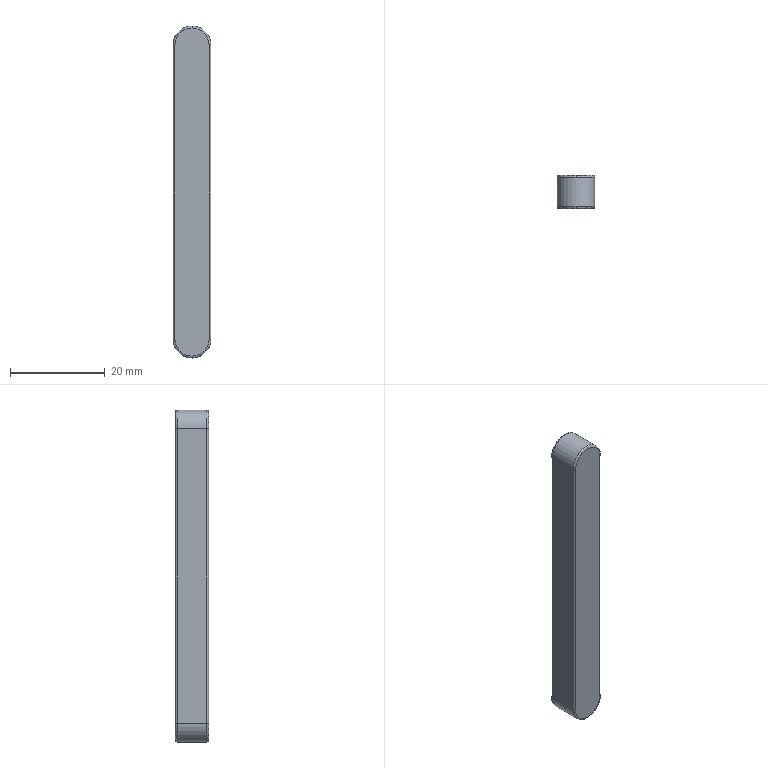Component | SolidWorks | ParallelKey4_70-1 | 1 solid | 17 faces | box 8 x 7 x 70 mm | volume 3814 mm3 | cylinder 7 | spline 6 | plane 4 | commonest cylinder face diameters 0.8 x4 8 x3
STEP:
#1=COLOUR_RGB('',0.7922,0.8196,0.9333);
#2=FILL_AREA_STYLE_COLOUR('',#1);
#3=FILL_AREA_STYLE('',(#2));
#4=SURFACE_STYLE_FILL_AREA(#3);
#5=SURFACE_SIDE_STYLE('',(#4));
#6=SURFACE_STYLE_USAGE(.BOTH.,#5);
#7=PRESENTATION_STYLE_ASSIGNMENT((#6));
#8=CARTESIAN_POINT('',(-12.421,-6.551,-9.22));
#9=VERTEX_POINT('',#8);
#10=CARTESIAN_POINT('',(-12.579,-6.551,-9.063));
#11=VERTEX_POINT('',#10);
#12=CARTESIAN_POINT('',(-12.579,-6.551,-9.22));
#13=DIRECTION('',(0.,-1.,0.));
#14=DIRECTION('',(0.,0.,1.));
#15=AXIS2_PLACEMENT_3D('',#12,#13,#14);
#16=CIRCLE('',#15,0.1575);
#17=EDGE_CURVE('',#9,#11,#16,.T.);
#18=ORIENTED_EDGE('',*,*,#17,.T.);
#19=CARTESIAN_POINT('',(-12.579,-6.567,-9.079));
#20=VERTEX_POINT('',#19);
#21=CARTESIAN_POINT('',(-12.579,-6.551,-9.079));
#22=DIRECTION('',(1.,0.,0.));
#23=DIRECTION('',(0.,0.,1.));
#24=AXIS2_PLACEMENT_3D('',#21,#22,#23);
#25=CIRCLE('',#24,0.01575);
#26=EDGE_CURVE('',#11,#20,#25,.T.);
#27=ORIENTED_EDGE('',*,*,#26,.T.);
#28=CARTESIAN_POINT('',(-12.437,-6.567,-9.22));
#29=VERTEX_POINT('',#28);
#30=CARTESIAN_POINT('',(-12.579,-6.567,-9.079));
#31=CARTESIAN_POINT('',(-12.496,-6.567,-9.079));
#32=CARTESIAN_POINT('',(-12.437,-6.567,-9.137));
#33=CARTESIAN_POINT('',(-12.437,-6.567,-9.22));
#34=(BOUNDED_CURVE()B_SPLINE_CURVE(3,(#30,#31,#32,#33),.UNSPECIFIED.,.F.,.F.)B_SPLINE_CURVE_WITH_KNOTS((4,4),(0.,1.),.UNSPECIFIED.)CURVE()GEOMETRIC_REPRESENTATION_ITEM()RATIONAL_B_SPLINE_CURVE((1.,0.8047,0.8047,1.))REPRESENTATION_ITEM(''));
#35=EDGE_CURVE('',#20,#29,#34,.T.);
#36=ORIENTED_EDGE('',*,*,#35,.T.);
#37=CARTESIAN_POINT('',(-12.437,-6.551,-9.22));
#38=DIRECTION('',(0.,0.,-1.));
#39=DIRECTION('',(-1.,0.,0.));
#40=AXIS2_PLACEMENT_3D('',#37,#38,#39);
#41=CIRCLE('',#40,0.01575);
#42=EDGE_CURVE('',#9,#29,#41,.T.);
#43=ORIENTED_EDGE('',*,*,#42,.F.);
#44=EDGE_LOOP('',(#18,#27,#36,#43));
#45=FACE_OUTER_BOUND('',#44,.T.);
#46=CARTESIAN_POINT('',(-12.579,-6.551,-9.063));
#47=CARTESIAN_POINT('',(-12.486,-6.551,-9.063));
#48=CARTESIAN_POINT('',(-12.421,-6.551,-9.128));
#49=CARTESIAN_POINT('',(-12.421,-6.551,-9.22));
#50=CARTESIAN_POINT('',(-12.579,-6.56,-9.063));
#51=CARTESIAN_POINT('',(-12.486,-6.56,-9.063));
#52=CARTESIAN_POINT('',(-12.421,-6.56,-9.128));
#53=CARTESIAN_POINT('',(-12.421,-6.56,-9.22));
#54=CARTESIAN_POINT('',(-12.579,-6.567,-9.07));
#55=CARTESIAN_POINT('',(-12.49,-6.567,-9.07));
#56=CARTESIAN_POINT('',(-12.428,-6.567,-9.132));
#57=CARTESIAN_POINT('',(-12.428,-6.567,-9.22));
#58=CARTESIAN_POINT('',(-12.579,-6.567,-9.079));
#59=CARTESIAN_POINT('',(-12.496,-6.567,-9.079));
#60=CARTESIAN_POINT('',(-12.437,-6.567,-9.137));
#61=CARTESIAN_POINT('',(-12.437,-6.567,-9.22));
#62=(BOUNDED_SURFACE()B_SPLINE_SURFACE(3,3,((#46,#47,#48,#49),(#50,#51,#52,#53),(#54,#55,#56,#57),(#58,#59,#60,#61)),.UNSPECIFIED.,.F.,.F.,.F.)B_SPLINE_SURFACE_WITH_KNOTS((4,4),(4,4),(0.,1.),(0.,1.),.UNSPECIFIED.)GEOMETRIC_REPRESENTATION_ITEM()RATIONAL_B_SPLINE_SURFACE(((1.,0.8047,0.8047,1.),(0.8047,0.6476,0.6476,0.8047),(0.8047,0.6476,0.6476,0.8047),(1.,0.8047,0.8047,1.)))REPRESENTATION_ITEM('')SURFACE());
#63=ADVANCED_FACE('',(#45),#62,.T.);
#64=CARTESIAN_POINT('',(-12.437,-6.291,-9.22));
#65=VERTEX_POINT('',#64);
#66=CARTESIAN_POINT('',(-12.579,-6.291,-9.079));
#67=VERTEX_POINT('',#66);
#68=CARTESIAN_POINT('',(-12.437,-6.291,-9.22));
#69=CARTESIAN_POINT('',(-12.437,-6.291,-9.137));
#70=CARTESIAN_POINT('',(-12.496,-6.291,-9.079));
#71=CARTESIAN_POINT('',(-12.579,-6.291,-9.079));
#72=(BOUNDED_CURVE()B_SPLINE_CURVE(3,(#68,#69,#70,#71),.UNSPECIFIED.,.F.,.F.)B_SPLINE_CURVE_WITH_KNOTS((4,4),(0.,1.),.UNSPECIFIED.)CURVE()GEOMETRIC_REPRESENTATION_ITEM()RATIONAL_B_SPLINE_CURVE((1.,0.8047,0.8047,1.))REPRESENTATION_ITEM(''));
#73=EDGE_CURVE('',#65,#67,#72,.T.);
#74=ORIENTED_EDGE('',*,*,#73,.T.);
#75=CARTESIAN_POINT('',(-12.579,-6.307,-9.063));
#76=VERTEX_POINT('',#75);
#77=CARTESIAN_POINT('',(-12.579,-6.307,-9.079));
#78=DIRECTION('',(1.,0.,0.));
#79=DIRECTION('',(0.,0.,1.));
#80=AXIS2_PLACEMENT_3D('',#77,#78,#79);
#81=CIRCLE('',#80,0.01575);
#82=EDGE_CURVE('',#67,#76,#81,.T.);
#83=ORIENTED_EDGE('',*,*,#82,.T.);
#84=CARTESIAN_POINT('',(-12.421,-6.307,-9.22));
#85=VERTEX_POINT('',#84);
#86=CARTESIAN_POINT('',(-12.579,-6.307,-9.22));
#87=DIRECTION('',(0.,-1.,0.));
#88=DIRECTION('',(0.,0.,-1.));
#89=AXIS2_PLACEMENT_3D('',#86,#87,#88);
#90=CIRCLE('',#89,0.1575);
#91=EDGE_CURVE('',#85,#76,#90,.T.);
#92=ORIENTED_EDGE('',*,*,#91,.F.);
#93=CARTESIAN_POINT('',(-12.437,-6.307,-9.22));
#94=DIRECTION('',(0.,0.,-1.));
#95=DIRECTION('',(1.,0.,0.));
#96=AXIS2_PLACEMENT_3D('',#93,#94,#95);
#97=CIRCLE('',#96,0.01575);
#98=EDGE_CURVE('',#65,#85,#97,.T.);
#99=ORIENTED_EDGE('',*,*,#98,.F.);
#100=EDGE_LOOP('',(#74,#83,#92,#99));
#101=FACE_OUTER_BOUND('',#100,.T.);
#102=CARTESIAN_POINT('',(-12.579,-6.291,-9.079));
#103=CARTESIAN_POINT('',(-12.496,-6.291,-9.079));
#104=CARTESIAN_POINT('',(-12.437,-6.291,-9.137));
#105=CARTESIAN_POINT('',(-12.437,-6.291,-9.22));
#106=CARTESIAN_POINT('',(-12.579,-6.291,-9.07));
#107=CARTESIAN_POINT('',(-12.49,-6.291,-9.07));
#108=CARTESIAN_POINT('',(-12.428,-6.291,-9.132));
#109=CARTESIAN_POINT('',(-12.428,-6.291,-9.22));
#110=CARTESIAN_POINT('',(-12.579,-6.298,-9.063));
#111=CARTESIAN_POINT('',(-12.486,-6.298,-9.063));
#112=CARTESIAN_POINT('',(-12.421,-6.298,-9.128));
#113=CARTESIAN_POINT('',(-12.421,-6.298,-9.22));
#114=CARTESIAN_POINT('',(-12.579,-6.307,-9.063));
#115=CARTESIAN_POINT('',(-12.486,-6.307,-9.063));
#116=CARTESIAN_POINT('',(-12.421,-6.307,-9.128));
#117=CARTESIAN_POINT('',(-12.421,-6.307,-9.22));
#118=(BOUNDED_SURFACE()B_SPLINE_SURFACE(3,3,((#102,#103,#104,#105),(#106,#107,#108,#109),(#110,#111,#112,#113),(#114,#115,#116,#117)),.UNSPECIFIED.,.F.,.F.,.F.)B_SPLINE_SURFACE_WITH_KNOTS((4,4),(4,4),(0.,1.),(0.,1.),.UNSPECIFIED.)GEOMETRIC_REPRESENTATION_ITEM()RATIONAL_B_SPLINE_SURFACE(((1.,0.8047,0.8047,1.),(0.8047,0.6476,0.6476,0.8047),(0.8047,0.6476,0.6476,0.8047),(1.,0.8047,0.8047,1.)))REPRESENTATION_ITEM('')SURFACE());
#119=ADVANCED_FACE('',(#101),#118,.T.);
#120=CARTESIAN_POINT('',(-12.736,-6.307,-11.661));
#121=VERTEX_POINT('',#120);
#122=CARTESIAN_POINT('',(-12.579,-6.307,-11.819));
#123=VERTEX_POINT('',#122);
#124=CARTESIAN_POINT('',(-12.579,-6.307,-11.661));
#125=DIRECTION('',(0.,-1.,0.));
#126=DIRECTION('',(0.,0.,-1.));
#127=AXIS2_PLACEMENT_3D('',#124,#125,#126);
#128=CIRCLE('',#127,0.1575);
#129=EDGE_CURVE('',#121,#123,#128,.T.);
#130=ORIENTED_EDGE('',*,*,#129,.T.);
#131=CARTESIAN_POINT('',(-12.579,-6.551,-11.819));
#132=VERTEX_POINT('',#131);
#133=CARTESIAN_POINT('',(-12.579,-6.291,-11.819));
#134=DIRECTION('',(0.,-1.,0.));
#135=VECTOR('',#134,39.37);
#136=LINE('',#133,#135);
#137=EDGE_CURVE('',#123,#132,#136,.T.);
#138=ORIENTED_EDGE('',*,*,#137,.T.);
#139=CARTESIAN_POINT('',(-12.736,-6.551,-11.661));
#140=VERTEX_POINT('',#139);
#141=CARTESIAN_POINT('',(-12.579,-6.551,-11.661));
#142=DIRECTION('',(0.,-1.,0.));
#143=DIRECTION('',(0.,0.,1.));
#144=AXIS2_PLACEMENT_3D('',#141,#142,#143);
#145=CIRCLE('',#144,0.1575);
#146=EDGE_CURVE('',#140,#132,#145,.T.);
#147=ORIENTED_EDGE('',*,*,#146,.F.);
#148=CARTESIAN_POINT('',(-12.736,-6.291,-11.661));
#149=DIRECTION('',(0.,1.,0.));
#150=VECTOR('',#149,39.37);
#151=LINE('',#148,#150);
#152=EDGE_CURVE('',#140,#121,#151,.T.);
#153=ORIENTED_EDGE('',*,*,#152,.T.);
#154=EDGE_LOOP('',(#130,#138,#147,#153));
#155=FACE_OUTER_BOUND('',#154,.T.);
#156=CARTESIAN_POINT('',(-12.579,-6.291,-11.661));
#157=DIRECTION('',(0.,-1.,0.));
#158=DIRECTION('',(0.,0.,-1.));
#159=AXIS2_PLACEMENT_3D('',#156,#157,#158);
#160=CYLINDRICAL_SURFACE('',#159,0.1575);
#161=ADVANCED_FACE('',(#155),#160,.T.);
#162=ORIENTED_EDGE('',*,*,#35,.F.);
#163=CARTESIAN_POINT('',(-12.72,-6.567,-9.22));
#164=VERTEX_POINT('',#163);
#165=CARTESIAN_POINT('',(-12.72,-6.567,-9.22));
#166=CARTESIAN_POINT('',(-12.72,-6.567,-9.137));
#167=CARTESIAN_POINT('',(-12.662,-6.567,-9.079));
#168=CARTESIAN_POINT('',(-12.579,-6.567,-9.079));
#169=(BOUNDED_CURVE()B_SPLINE_CURVE(3,(#165,#166,#167,#168),.UNSPECIFIED.,.F.,.T.)B_SPLINE_CURVE_WITH_KNOTS((4,4),(0.,1.),.UNSPECIFIED.)CURVE()GEOMETRIC_REPRESENTATION_ITEM()RATIONAL_B_SPLINE_CURVE((1.,0.8047,0.8047,1.))REPRESENTATION_ITEM(''));
#170=EDGE_CURVE('',#164,#20,#169,.T.);
#171=ORIENTED_EDGE('',*,*,#170,.F.);
#172=CARTESIAN_POINT('',(-12.72,-6.567,-11.661));
#173=VERTEX_POINT('',#172);
#174=CARTESIAN_POINT('',(-12.72,-6.567,-11.661));
#175=DIRECTION('',(-0.,0.,1.));
#176=VECTOR('',#175,39.37);
#177=LINE('',#174,#176);
#178=EDGE_CURVE('',#173,#164,#177,.T.);
#179=ORIENTED_EDGE('',*,*,#178,.F.);
#180=CARTESIAN_POINT('',(-12.437,-6.567,-11.661));
#181=VERTEX_POINT('',#180);
#182=CARTESIAN_POINT('',(-12.437,-6.567,-11.661));
#183=CARTESIAN_POINT('',(-12.437,-6.567,-11.945));
#184=CARTESIAN_POINT('',(-12.72,-6.567,-11.945));
#185=CARTESIAN_POINT('',(-12.72,-6.567,-11.661));
#186=(BOUNDED_CURVE()B_SPLINE_CURVE(3,(#182,#183,#184,#185),.UNSPECIFIED.,.F.,.F.)B_SPLINE_CURVE_WITH_KNOTS((4,4),(0.,1.),.UNSPECIFIED.)CURVE()GEOMETRIC_REPRESENTATION_ITEM()RATIONAL_B_SPLINE_CURVE((1.,0.3333,0.3333,1.))REPRESENTATION_ITEM(''));
#187=EDGE_CURVE('',#181,#173,#186,.T.);
#188=ORIENTED_EDGE('',*,*,#187,.F.);
#189=CARTESIAN_POINT('',(-12.437,-6.567,-11.661));
#190=DIRECTION('',(0.,0.,-1.));
#191=VECTOR('',#190,39.37);
#192=LINE('',#189,#191);
#193=EDGE_CURVE('',#29,#181,#192,.T.);
#194=ORIENTED_EDGE('',*,*,#193,.F.);
#195=EDGE_LOOP('',(#162,#171,#179,#188,#194));
#196=FACE_OUTER_BOUND('',#195,.T.);
#197=CARTESIAN_POINT('',(-12.579,-6.567,-11.661));
#198=DIRECTION('',(0.,1.,0.));
#199=DIRECTION('',(-0.,0.,1.));
#200=AXIS2_PLACEMENT_3D('',#197,#198,#199);
#201=PLANE('',#200);
#202=ADVANCED_FACE('',(#196),#201,.F.);
#203=ORIENTED_EDGE('',*,*,#42,.T.);
#204=ORIENTED_EDGE('',*,*,#193,.T.);
#205=CARTESIAN_POINT('',(-12.421,-6.551,-11.661));
#206=VERTEX_POINT('',#205);
#207=CARTESIAN_POINT('',(-12.437,-6.551,-11.661));
#208=DIRECTION('',(0.,0.,1.));
#209=DIRECTION('',(-1.,0.,0.));
#210=AXIS2_PLACEMENT_3D('',#207,#208,#209);
#211=CIRCLE('',#210,0.01575);
#212=EDGE_CURVE('',#181,#206,#211,.T.);
#213=ORIENTED_EDGE('',*,*,#212,.T.);
#214=CARTESIAN_POINT('',(-12.421,-6.551,-11.661));
#215=DIRECTION('',(0.,0.,1.));
#216=VECTOR('',#215,39.37);
#217=LINE('',#214,#216);
#218=EDGE_CURVE('',#206,#9,#217,.T.);
#219=ORIENTED_EDGE('',*,*,#218,.T.);
#220=EDGE_LOOP('',(#203,#204,#213,#219));
#221=FACE_OUTER_BOUND('',#220,.T.);
#222=CARTESIAN_POINT('',(-12.437,-6.551,-11.661));
#223=DIRECTION('',(0.,0.,-1.));
#224=DIRECTION('',(-1.,0.,0.));
#225=AXIS2_PLACEMENT_3D('',#222,#223,#224);
#226=CYLINDRICAL_SURFACE('',#225,0.01575);
#227=ADVANCED_FACE('',(#221),#226,.T.);
#228=ORIENTED_EDGE('',*,*,#26,.F.);
#229=CARTESIAN_POINT('',(-12.736,-6.551,-9.22));
#230=VERTEX_POINT('',#229);
#231=CARTESIAN_POINT('',(-12.579,-6.551,-9.22));
#232=DIRECTION('',(0.,-1.,0.));
#233=DIRECTION('',(0.,0.,1.));
#234=AXIS2_PLACEMENT_3D('',#231,#232,#233);
#235=CIRCLE('',#234,0.1575);
#236=EDGE_CURVE('',#11,#230,#235,.T.);
#237=ORIENTED_EDGE('',*,*,#236,.T.);
#238=CARTESIAN_POINT('',(-12.72,-6.551,-9.22));
#239=DIRECTION('',(-0.,0.,1.));
#240=DIRECTION('',(-1.,0.,0.));
#241=AXIS2_PLACEMENT_3D('',#238,#239,#240);
#242=CIRCLE('',#241,0.01575);
#243=EDGE_CURVE('',#230,#164,#242,.T.);
#244=ORIENTED_EDGE('',*,*,#243,.T.);
#245=ORIENTED_EDGE('',*,*,#170,.T.);
#246=EDGE_LOOP('',(#228,#237,#244,#245));
#247=FACE_OUTER_BOUND('',#246,.T.);
#248=CARTESIAN_POINT('',(-12.736,-6.551,-9.22));
#249=CARTESIAN_POINT('',(-12.736,-6.551,-9.128));
#250=CARTESIAN_POINT('',(-12.671,-6.551,-9.063));
#251=CARTESIAN_POINT('',(-12.579,-6.551,-9.063));
#252=CARTESIAN_POINT('',(-12.736,-6.56,-9.22));
#253=CARTESIAN_POINT('',(-12.736,-6.56,-9.128));
#254=CARTESIAN_POINT('',(-12.671,-6.56,-9.063));
#255=CARTESIAN_POINT('',(-12.579,-6.56,-9.063));
#256=CARTESIAN_POINT('',(-12.73,-6.567,-9.22));
#257=CARTESIAN_POINT('',(-12.73,-6.567,-9.132));
#258=CARTESIAN_POINT('',(-12.667,-6.567,-9.07));
#259=CARTESIAN_POINT('',(-12.579,-6.567,-9.07));
#260=CARTESIAN_POINT('',(-12.72,-6.567,-9.22));
#261=CARTESIAN_POINT('',(-12.72,-6.567,-9.137));
#262=CARTESIAN_POINT('',(-12.662,-6.567,-9.079));
#263=CARTESIAN_POINT('',(-12.579,-6.567,-9.079));
#264=(BOUNDED_SURFACE()B_SPLINE_SURFACE(3,3,((#248,#249,#250,#251),(#252,#253,#254,#255),(#256,#257,#258,#259),(#260,#261,#262,#263)),.UNSPECIFIED.,.F.,.F.,.T.)B_SPLINE_SURFACE_WITH_KNOTS((4,4),(4,4),(0.,1.),(0.,1.),.UNSPECIFIED.)GEOMETRIC_REPRESENTATION_ITEM()RATIONAL_B_SPLINE_SURFACE(((1.,0.8047,0.8047,1.),(0.8047,0.6476,0.6476,0.8047),(0.8047,0.6476,0.6476,0.8047),(1.,0.8047,0.8047,1.)))REPRESENTATION_ITEM('')SURFACE());
#265=ADVANCED_FACE('',(#247),#264,.T.);
#266=ORIENTED_EDGE('',*,*,#243,.F.);
#267=CARTESIAN_POINT('',(-12.736,-6.551,-11.661));
#268=DIRECTION('',(0.,0.,-1.));
#269=VECTOR('',#268,39.37);
#270=LINE('',#267,#269);
#271=EDGE_CURVE('',#230,#140,#270,.T.);
#272=ORIENTED_EDGE('',*,*,#271,.T.);
#273=CARTESIAN_POINT('',(-12.72,-6.551,-11.661));
#274=DIRECTION('',(-0.,0.,1.));
#275=DIRECTION('',(1.,0.,0.));
#276=AXIS2_PLACEMENT_3D('',#273,#274,#275);
#277=CIRCLE('',#276,0.01575);
#278=EDGE_CURVE('',#140,#173,#277,.T.);
#279=ORIENTED_EDGE('',*,*,#278,.T.);
#280=ORIENTED_EDGE('',*,*,#178,.T.);
#281=EDGE_LOOP('',(#266,#272,#279,#280));
#282=FACE_OUTER_BOUND('',#281,.T.);
#283=CARTESIAN_POINT('',(-12.72,-6.551,-11.661));
#284=DIRECTION('',(-0.,0.,1.));
#285=DIRECTION('',(1.,0.,0.));
#286=AXIS2_PLACEMENT_3D('',#283,#284,#285);
#287=CYLINDRICAL_SURFACE('',#286,0.01575);
#288=ADVANCED_FACE('',(#282),#287,.T.);
#289=ORIENTED_EDGE('',*,*,#278,.F.);
#290=ORIENTED_EDGE('',*,*,#146,.T.);
#291=CARTESIAN_POINT('',(-12.579,-6.551,-11.661));
#292=DIRECTION('',(0.,-1.,0.));
#293=DIRECTION('',(0.,0.,1.));
#294=AXIS2_PLACEMENT_3D('',#291,#292,#293);
#295=CIRCLE('',#294,0.1575);
#296=EDGE_CURVE('',#132,#206,#295,.T.);
#297=ORIENTED_EDGE('',*,*,#296,.T.);
#298=ORIENTED_EDGE('',*,*,#212,.F.);
#299=ORIENTED_EDGE('',*,*,#187,.T.);
#300=EDGE_LOOP('',(#289,#290,#297,#298,#299));
#301=FACE_OUTER_BOUND('',#300,.T.);
#302=CARTESIAN_POINT('',(-12.421,-6.551,-11.661));
#303=CARTESIAN_POINT('',(-12.421,-6.551,-11.976));
#304=CARTESIAN_POINT('',(-12.736,-6.551,-11.976));
#305=CARTESIAN_POINT('',(-12.736,-6.551,-11.661));
#306=CARTESIAN_POINT('',(-12.421,-6.56,-11.661));
#307=CARTESIAN_POINT('',(-12.421,-6.56,-11.976));
#308=CARTESIAN_POINT('',(-12.736,-6.56,-11.976));
#309=CARTESIAN_POINT('',(-12.736,-6.56,-11.661));
#310=CARTESIAN_POINT('',(-12.428,-6.567,-11.661));
#311=CARTESIAN_POINT('',(-12.428,-6.567,-11.963));
#312=CARTESIAN_POINT('',(-12.73,-6.567,-11.963));
#313=CARTESIAN_POINT('',(-12.73,-6.567,-11.661));
#314=CARTESIAN_POINT('',(-12.437,-6.567,-11.661));
#315=CARTESIAN_POINT('',(-12.437,-6.567,-11.945));
#316=CARTESIAN_POINT('',(-12.72,-6.567,-11.945));
#317=CARTESIAN_POINT('',(-12.72,-6.567,-11.661));
#318=(BOUNDED_SURFACE()B_SPLINE_SURFACE(3,3,((#302,#303,#304,#305),(#306,#307,#308,#309),(#310,#311,#312,#313),(#314,#315,#316,#317)),.UNSPECIFIED.,.F.,.F.,.T.)B_SPLINE_SURFACE_WITH_KNOTS((4,4),(4,4),(0.,1.),(0.,1.),.UNSPECIFIED.)GEOMETRIC_REPRESENTATION_ITEM()RATIONAL_B_SPLINE_SURFACE(((1.,0.3333,0.3333,1.),(0.8047,0.2682,0.2682,0.8047),(0.8047,0.2682,0.2682,0.8047),(1.,0.3333,0.3333,1.)))REPRESENTATION_ITEM('')SURFACE());
#319=ADVANCED_FACE('',(#301),#318,.T.);
#320=CARTESIAN_POINT('',(-12.421,-6.307,-11.661));
#321=VERTEX_POINT('',#320);
#322=CARTESIAN_POINT('',(-12.421,-6.307,-11.661));
#323=DIRECTION('',(0.,0.,-1.));
#324=VECTOR('',#323,39.37);
#325=LINE('',#322,#324);
#326=EDGE_CURVE('',#85,#321,#325,.T.);
#327=ORIENTED_EDGE('',*,*,#326,.F.);
#328=CARTESIAN_POINT('',(-12.421,-6.291,-9.22));
#329=DIRECTION('',(0.,1.,0.));
#330=VECTOR('',#329,39.37);
#331=LINE('',#328,#330);
#332=EDGE_CURVE('',#9,#85,#331,.T.);
#333=ORIENTED_EDGE('',*,*,#332,.F.);
#334=ORIENTED_EDGE('',*,*,#218,.F.);
#335=CARTESIAN_POINT('',(-12.421,-6.291,-11.661));
#336=DIRECTION('',(0.,-1.,0.));
#337=VECTOR('',#336,39.37);
#338=LINE('',#335,#337);
#339=EDGE_CURVE('',#321,#206,#338,.T.);
#340=ORIENTED_EDGE('',*,*,#339,.F.);
#341=EDGE_LOOP('',(#327,#333,#334,#340));
#342=FACE_OUTER_BOUND('',#341,.T.);
#343=CARTESIAN_POINT('',(-12.421,-6.291,-11.661));
#344=DIRECTION('',(-1.,0.,0.));
#345=DIRECTION('',(0.,0.,1.));
#346=AXIS2_PLACEMENT_3D('',#343,#344,#345);
#347=PLANE('',#346);
#348=ADVANCED_FACE('',(#342),#347,.F.);
#349=CARTESIAN_POINT('',(-12.736,-6.307,-9.22));
#350=VERTEX_POINT('',#349);
#351=CARTESIAN_POINT('',(-12.736,-6.291,-9.22));
#352=DIRECTION('',(0.,-1.,0.));
#353=VECTOR('',#352,39.37);
#354=LINE('',#351,#353);
#355=EDGE_CURVE('',#350,#230,#354,.T.);
#356=ORIENTED_EDGE('',*,*,#355,.T.);
#357=ORIENTED_EDGE('',*,*,#236,.F.);
#358=ORIENTED_EDGE('',*,*,#17,.F.);
#359=ORIENTED_EDGE('',*,*,#332,.T.);
#360=ORIENTED_EDGE('',*,*,#91,.T.);
#361=CARTESIAN_POINT('',(-12.579,-6.307,-9.22));
#362=DIRECTION('',(0.,-1.,0.));
#363=DIRECTION('',(0.,0.,-1.));
#364=AXIS2_PLACEMENT_3D('',#361,#362,#363);
#365=CIRCLE('',#364,0.1575);
#366=EDGE_CURVE('',#76,#350,#365,.T.);
#367=ORIENTED_EDGE('',*,*,#366,.T.);
#368=EDGE_LOOP('',(#356,#357,#358,#359,#360,#367));
#369=FACE_OUTER_BOUND('',#368,.T.);
#370=CARTESIAN_POINT('',(-12.579,-6.291,-9.22));
#371=DIRECTION('',(0.,-1.,0.));
#372=DIRECTION('',(0.,0.,-1.));
#373=AXIS2_PLACEMENT_3D('',#370,#371,#372);
#374=CYLINDRICAL_SURFACE('',#373,0.1575);
#375=ADVANCED_FACE('',(#369),#374,.T.);
#376=CARTESIAN_POINT('',(-12.736,-6.307,-11.661));
#377=DIRECTION('',(-0.,0.,1.));
#378=VECTOR('',#377,39.37);
#379=LINE('',#376,#378);
#380=EDGE_CURVE('',#121,#350,#379,.T.);
#381=ORIENTED_EDGE('',*,*,#380,.F.);
#382=ORIENTED_EDGE('',*,*,#152,.F.);
#383=ORIENTED_EDGE('',*,*,#271,.F.);
#384=ORIENTED_EDGE('',*,*,#355,.F.);
#385=EDGE_LOOP('',(#381,#382,#383,#384));
#386=FACE_OUTER_BOUND('',#385,.T.);
#387=CARTESIAN_POINT('',(-12.736,-6.291,-11.661));
#388=DIRECTION('',(1.,0.,0.));
#389=DIRECTION('',(0.,0.,-1.));
#390=AXIS2_PLACEMENT_3D('',#387,#388,#389);
#391=PLANE('',#390);
#392=ADVANCED_FACE('',(#386),#391,.F.);
#393=ORIENTED_EDGE('',*,*,#137,.F.);
#394=CARTESIAN_POINT('',(-12.579,-6.307,-11.661));
#395=DIRECTION('',(0.,-1.,0.));
#396=DIRECTION('',(0.,0.,-1.));
#397=AXIS2_PLACEMENT_3D('',#394,#395,#396);
#398=CIRCLE('',#397,0.1575);
#399=EDGE_CURVE('',#123,#321,#398,.T.);
#400=ORIENTED_EDGE('',*,*,#399,.T.);
#401=ORIENTED_EDGE('',*,*,#339,.T.);
#402=ORIENTED_EDGE('',*,*,#296,.F.);
#403=EDGE_LOOP('',(#393,#400,#401,#402));
#404=FACE_OUTER_BOUND('',#403,.T.);
#405=CARTESIAN_POINT('',(-12.579,-6.291,-11.661));
#406=DIRECTION('',(0.,-1.,0.));
#407=DIRECTION('',(0.,0.,-1.));
#408=AXIS2_PLACEMENT_3D('',#405,#406,#407);
#409=CYLINDRICAL_SURFACE('',#408,0.1575);
#410=ADVANCED_FACE('',(#404),#409,.T.);
#411=ORIENTED_EDGE('',*,*,#98,.T.);
#412=ORIENTED_EDGE('',*,*,#326,.T.);
#413=CARTESIAN_POINT('',(-12.437,-6.291,-11.661));
#414=VERTEX_POINT('',#413);
#415=CARTESIAN_POINT('',(-12.437,-6.307,-11.661));
#416=DIRECTION('',(0.,0.,1.));
#417=DIRECTION('',(1.,0.,0.));
#418=AXIS2_PLACEMENT_3D('',#415,#416,#417);
#419=CIRCLE('',#418,0.01575);
#420=EDGE_CURVE('',#321,#414,#419,.T.);
#421=ORIENTED_EDGE('',*,*,#420,.T.);
#422=CARTESIAN_POINT('',(-12.437,-6.291,-11.661));
#423=DIRECTION('',(0.,0.,1.));
#424=VECTOR('',#423,39.37);
#425=LINE('',#422,#424);
#426=EDGE_CURVE('',#414,#65,#425,.T.);
#427=ORIENTED_EDGE('',*,*,#426,.T.);
#428=EDGE_LOOP('',(#411,#412,#421,#427));
#429=FACE_OUTER_BOUND('',#428,.T.);
#430=CARTESIAN_POINT('',(-12.437,-6.307,-11.661));
#431=DIRECTION('',(0.,0.,1.));
#432=DIRECTION('',(1.,0.,0.));
#433=AXIS2_PLACEMENT_3D('',#430,#431,#432);
#434=CYLINDRICAL_SURFACE('',#433,0.01575);
#435=ADVANCED_FACE('',(#429),#434,.T.);
#436=ORIENTED_EDGE('',*,*,#82,.F.);
#437=CARTESIAN_POINT('',(-12.72,-6.291,-9.22));
#438=VERTEX_POINT('',#437);
#439=CARTESIAN_POINT('',(-12.579,-6.291,-9.079));
#440=CARTESIAN_POINT('',(-12.662,-6.291,-9.079));
#441=CARTESIAN_POINT('',(-12.72,-6.291,-9.137));
#442=CARTESIAN_POINT('',(-12.72,-6.291,-9.22));
#443=(BOUNDED_CURVE()B_SPLINE_CURVE(3,(#439,#440,#441,#442),.UNSPECIFIED.,.F.,.F.)B_SPLINE_CURVE_WITH_KNOTS((4,4),(0.,1.),.UNSPECIFIED.)CURVE()GEOMETRIC_REPRESENTATION_ITEM()RATIONAL_B_SPLINE_CURVE((1.,0.8047,0.8047,1.))REPRESENTATION_ITEM(''));
#444=EDGE_CURVE('',#67,#438,#443,.T.);
#445=ORIENTED_EDGE('',*,*,#444,.T.);
#446=CARTESIAN_POINT('',(-12.72,-6.307,-9.22));
#447=DIRECTION('',(-0.,0.,1.));
#448=DIRECTION('',(-1.,0.,0.));
#449=AXIS2_PLACEMENT_3D('',#446,#447,#448);
#450=CIRCLE('',#449,0.01575);
#451=EDGE_CURVE('',#438,#350,#450,.T.);
#452=ORIENTED_EDGE('',*,*,#451,.T.);
#453=ORIENTED_EDGE('',*,*,#366,.F.);
#454=EDGE_LOOP('',(#436,#445,#452,#453));
#455=FACE_OUTER_BOUND('',#454,.T.);
#456=CARTESIAN_POINT('',(-12.72,-6.291,-9.22));
#457=CARTESIAN_POINT('',(-12.72,-6.291,-9.137));
#458=CARTESIAN_POINT('',(-12.662,-6.291,-9.079));
#459=CARTESIAN_POINT('',(-12.579,-6.291,-9.079));
#460=CARTESIAN_POINT('',(-12.73,-6.291,-9.22));
#461=CARTESIAN_POINT('',(-12.73,-6.291,-9.132));
#462=CARTESIAN_POINT('',(-12.667,-6.291,-9.07));
#463=CARTESIAN_POINT('',(-12.579,-6.291,-9.07));
#464=CARTESIAN_POINT('',(-12.736,-6.298,-9.22));
#465=CARTESIAN_POINT('',(-12.736,-6.298,-9.128));
#466=CARTESIAN_POINT('',(-12.671,-6.298,-9.063));
#467=CARTESIAN_POINT('',(-12.579,-6.298,-9.063));
#468=CARTESIAN_POINT('',(-12.736,-6.307,-9.22));
#469=CARTESIAN_POINT('',(-12.736,-6.307,-9.128));
#470=CARTESIAN_POINT('',(-12.671,-6.307,-9.063));
#471=CARTESIAN_POINT('',(-12.579,-6.307,-9.063));
#472=(BOUNDED_SURFACE()B_SPLINE_SURFACE(3,3,((#456,#457,#458,#459),(#460,#461,#462,#463),(#464,#465,#466,#467),(#468,#469,#470,#471)),.UNSPECIFIED.,.F.,.F.,.T.)B_SPLINE_SURFACE_WITH_KNOTS((4,4),(4,4),(0.,1.),(0.,1.),.UNSPECIFIED.)GEOMETRIC_REPRESENTATION_ITEM()RATIONAL_B_SPLINE_SURFACE(((1.,0.8047,0.8047,1.),(0.8047,0.6476,0.6476,0.8047),(0.8047,0.6476,0.6476,0.8047),(1.,0.8047,0.8047,1.)))REPRESENTATION_ITEM('')SURFACE());
#473=ADVANCED_FACE('',(#455),#472,.T.);
#474=ORIENTED_EDGE('',*,*,#451,.F.);
#475=CARTESIAN_POINT('',(-12.72,-6.291,-11.661));
#476=VERTEX_POINT('',#475);
#477=CARTESIAN_POINT('',(-12.72,-6.291,-11.661));
#478=DIRECTION('',(0.,0.,-1.));
#479=VECTOR('',#478,39.37);
#480=LINE('',#477,#479);
#481=EDGE_CURVE('',#438,#476,#480,.T.);
#482=ORIENTED_EDGE('',*,*,#481,.T.);
#483=CARTESIAN_POINT('',(-12.72,-6.307,-11.661));
#484=DIRECTION('',(-0.,0.,1.));
#485=DIRECTION('',(-1.,0.,0.));
#486=AXIS2_PLACEMENT_3D('',#483,#484,#485);
#487=CIRCLE('',#486,0.01575);
#488=EDGE_CURVE('',#476,#121,#487,.T.);
#489=ORIENTED_EDGE('',*,*,#488,.T.);
#490=ORIENTED_EDGE('',*,*,#380,.T.);
#491=EDGE_LOOP('',(#474,#482,#489,#490));
#492=FACE_OUTER_BOUND('',#491,.T.);
#493=CARTESIAN_POINT('',(-12.72,-6.307,-11.661));
#494=DIRECTION('',(0.,0.,-1.));
#495=DIRECTION('',(-1.,0.,0.));
#496=AXIS2_PLACEMENT_3D('',#493,#494,#495);
#497=CYLINDRICAL_SURFACE('',#496,0.01575);
#498=ADVANCED_FACE('',(#492),#497,.T.);
#499=ORIENTED_EDGE('',*,*,#488,.F.);
#500=CARTESIAN_POINT('',(-12.72,-6.291,-11.661));
#501=CARTESIAN_POINT('',(-12.72,-6.291,-11.945));
#502=CARTESIAN_POINT('',(-12.437,-6.291,-11.945));
#503=CARTESIAN_POINT('',(-12.437,-6.291,-11.661));
#504=(BOUNDED_CURVE()B_SPLINE_CURVE(3,(#500,#501,#502,#503),.UNSPECIFIED.,.F.,.F.)B_SPLINE_CURVE_WITH_KNOTS((4,4),(0.,1.),.UNSPECIFIED.)CURVE()GEOMETRIC_REPRESENTATION_ITEM()RATIONAL_B_SPLINE_CURVE((1.,0.3333,0.3333,1.))REPRESENTATION_ITEM(''));
#505=EDGE_CURVE('',#476,#414,#504,.T.);
#506=ORIENTED_EDGE('',*,*,#505,.T.);
#507=ORIENTED_EDGE('',*,*,#420,.F.);
#508=ORIENTED_EDGE('',*,*,#399,.F.);
#509=ORIENTED_EDGE('',*,*,#129,.F.);
#510=EDGE_LOOP('',(#499,#506,#507,#508,#509));
#511=FACE_OUTER_BOUND('',#510,.T.);
#512=CARTESIAN_POINT('',(-12.437,-6.291,-11.661));
#513=CARTESIAN_POINT('',(-12.437,-6.291,-11.945));
#514=CARTESIAN_POINT('',(-12.72,-6.291,-11.945));
#515=CARTESIAN_POINT('',(-12.72,-6.291,-11.661));
#516=CARTESIAN_POINT('',(-12.428,-6.291,-11.661));
#517=CARTESIAN_POINT('',(-12.428,-6.291,-11.963));
#518=CARTESIAN_POINT('',(-12.73,-6.291,-11.963));
#519=CARTESIAN_POINT('',(-12.73,-6.291,-11.661));
#520=CARTESIAN_POINT('',(-12.421,-6.298,-11.661));
#521=CARTESIAN_POINT('',(-12.421,-6.298,-11.976));
#522=CARTESIAN_POINT('',(-12.736,-6.298,-11.976));
#523=CARTESIAN_POINT('',(-12.736,-6.298,-11.661));
#524=CARTESIAN_POINT('',(-12.421,-6.307,-11.661));
#525=CARTESIAN_POINT('',(-12.421,-6.307,-11.976));
#526=CARTESIAN_POINT('',(-12.736,-6.307,-11.976));
#527=CARTESIAN_POINT('',(-12.736,-6.307,-11.661));
#528=(BOUNDED_SURFACE()B_SPLINE_SURFACE(3,3,((#512,#513,#514,#515),(#516,#517,#518,#519),(#520,#521,#522,#523),(#524,#525,#526,#527)),.UNSPECIFIED.,.F.,.F.,.T.)B_SPLINE_SURFACE_WITH_KNOTS((4,4),(4,4),(0.,1.),(0.,1.),.UNSPECIFIED.)GEOMETRIC_REPRESENTATION_ITEM()RATIONAL_B_SPLINE_SURFACE(((1.,0.3333,0.3333,1.),(0.8047,0.2682,0.2682,0.8047),(0.8047,0.2682,0.2682,0.8047),(1.,0.3333,0.3333,1.)))REPRESENTATION_ITEM('')SURFACE());
#529=ADVANCED_FACE('',(#511),#528,.T.);
#530=ORIENTED_EDGE('',*,*,#426,.F.);
#531=ORIENTED_EDGE('',*,*,#505,.F.);
#532=ORIENTED_EDGE('',*,*,#481,.F.);
#533=ORIENTED_EDGE('',*,*,#444,.F.);
#534=ORIENTED_EDGE('',*,*,#73,.F.);
#535=EDGE_LOOP('',(#530,#531,#532,#533,#534));
#536=FACE_OUTER_BOUND('',#535,.T.);
#537=CARTESIAN_POINT('',(-12.579,-6.291,-11.661));
#538=DIRECTION('',(0.,1.,0.));
#539=DIRECTION('',(-0.,0.,1.));
#540=AXIS2_PLACEMENT_3D('',#537,#538,#539);
#541=PLANE('',#540);
#542=ADVANCED_FACE('',(#536),#541,.T.);
#543=CLOSED_SHELL('',(#63,#119,#161,#202,#227,#265,#288,#319,#348,#375,#392,#410,#435,#473,#498,#529,#542));
#544=MANIFOLD_SOLID_BREP('',#543);
#545=STYLED_ITEM('',(#7),#544);
#546=PRESENTATION_LAYER_ASSIGNMENT('','',(#545));
#547=(LENGTH_UNIT()NAMED_UNIT(*)SI_UNIT($,.METRE.));
#548=LENGTH_MEASURE_WITH_UNIT(LENGTH_MEASURE(0.0254),#547);
#549=DIMENSIONAL_EXPONENTS(1.,0.,0.,0.,0.,0.,0.);
#550=(CONVERSION_BASED_UNIT('',#548)LENGTH_UNIT()NAMED_UNIT(#549));
#551=UNCERTAINTY_MEASURE_WITH_UNIT(LENGTH_MEASURE(0.00001),#550,'','');
#552=(NAMED_UNIT(*)PLANE_ANGLE_UNIT()SI_UNIT($,.RADIAN.));
#553=(NAMED_UNIT(*)SI_UNIT($,.STERADIAN.)SOLID_ANGLE_UNIT());
#554=(GEOMETRIC_REPRESENTATION_CONTEXT(3)GLOBAL_UNCERTAINTY_ASSIGNED_CONTEXT((#551))GLOBAL_UNIT_ASSIGNED_CONTEXT((#550,#552,#553))REPRESENTATION_CONTEXT('',''));
#555=MECHANICAL_DESIGN_GEOMETRIC_PRESENTATION_REPRESENTATION('',(#545),#554);
#556=CARTESIAN_POINT('',(0.,0.,0.));
#557=DIRECTION('',(0.,0.,1.));
#558=DIRECTION('',(1.,0.,0.));
#559=AXIS2_PLACEMENT_3D('',#556,#557,#558);
#560=(LENGTH_UNIT()NAMED_UNIT(*)SI_UNIT($,.METRE.));
#561=LENGTH_MEASURE_WITH_UNIT(LENGTH_MEASURE(0.0254),#560);
#562=DIMENSIONAL_EXPONENTS(1.,0.,0.,0.,0.,0.,0.);
#563=(CONVERSION_BASED_UNIT('',#561)LENGTH_UNIT()NAMED_UNIT(#562));
#564=UNCERTAINTY_MEASURE_WITH_UNIT(LENGTH_MEASURE(0.00001),#563,'','');
#565=(NAMED_UNIT(*)PLANE_ANGLE_UNIT()SI_UNIT($,.RADIAN.));
#566=(NAMED_UNIT(*)SI_UNIT($,.STERADIAN.)SOLID_ANGLE_UNIT());
#567=(GEOMETRIC_REPRESENTATION_CONTEXT(3)GLOBAL_UNCERTAINTY_ASSIGNED_CONTEXT((#564))GLOBAL_UNIT_ASSIGNED_CONTEXT((#563,#565,#566))REPRESENTATION_CONTEXT('',''));
#568=ADVANCED_BREP_SHAPE_REPRESENTATION('',(#544,#559),#567);